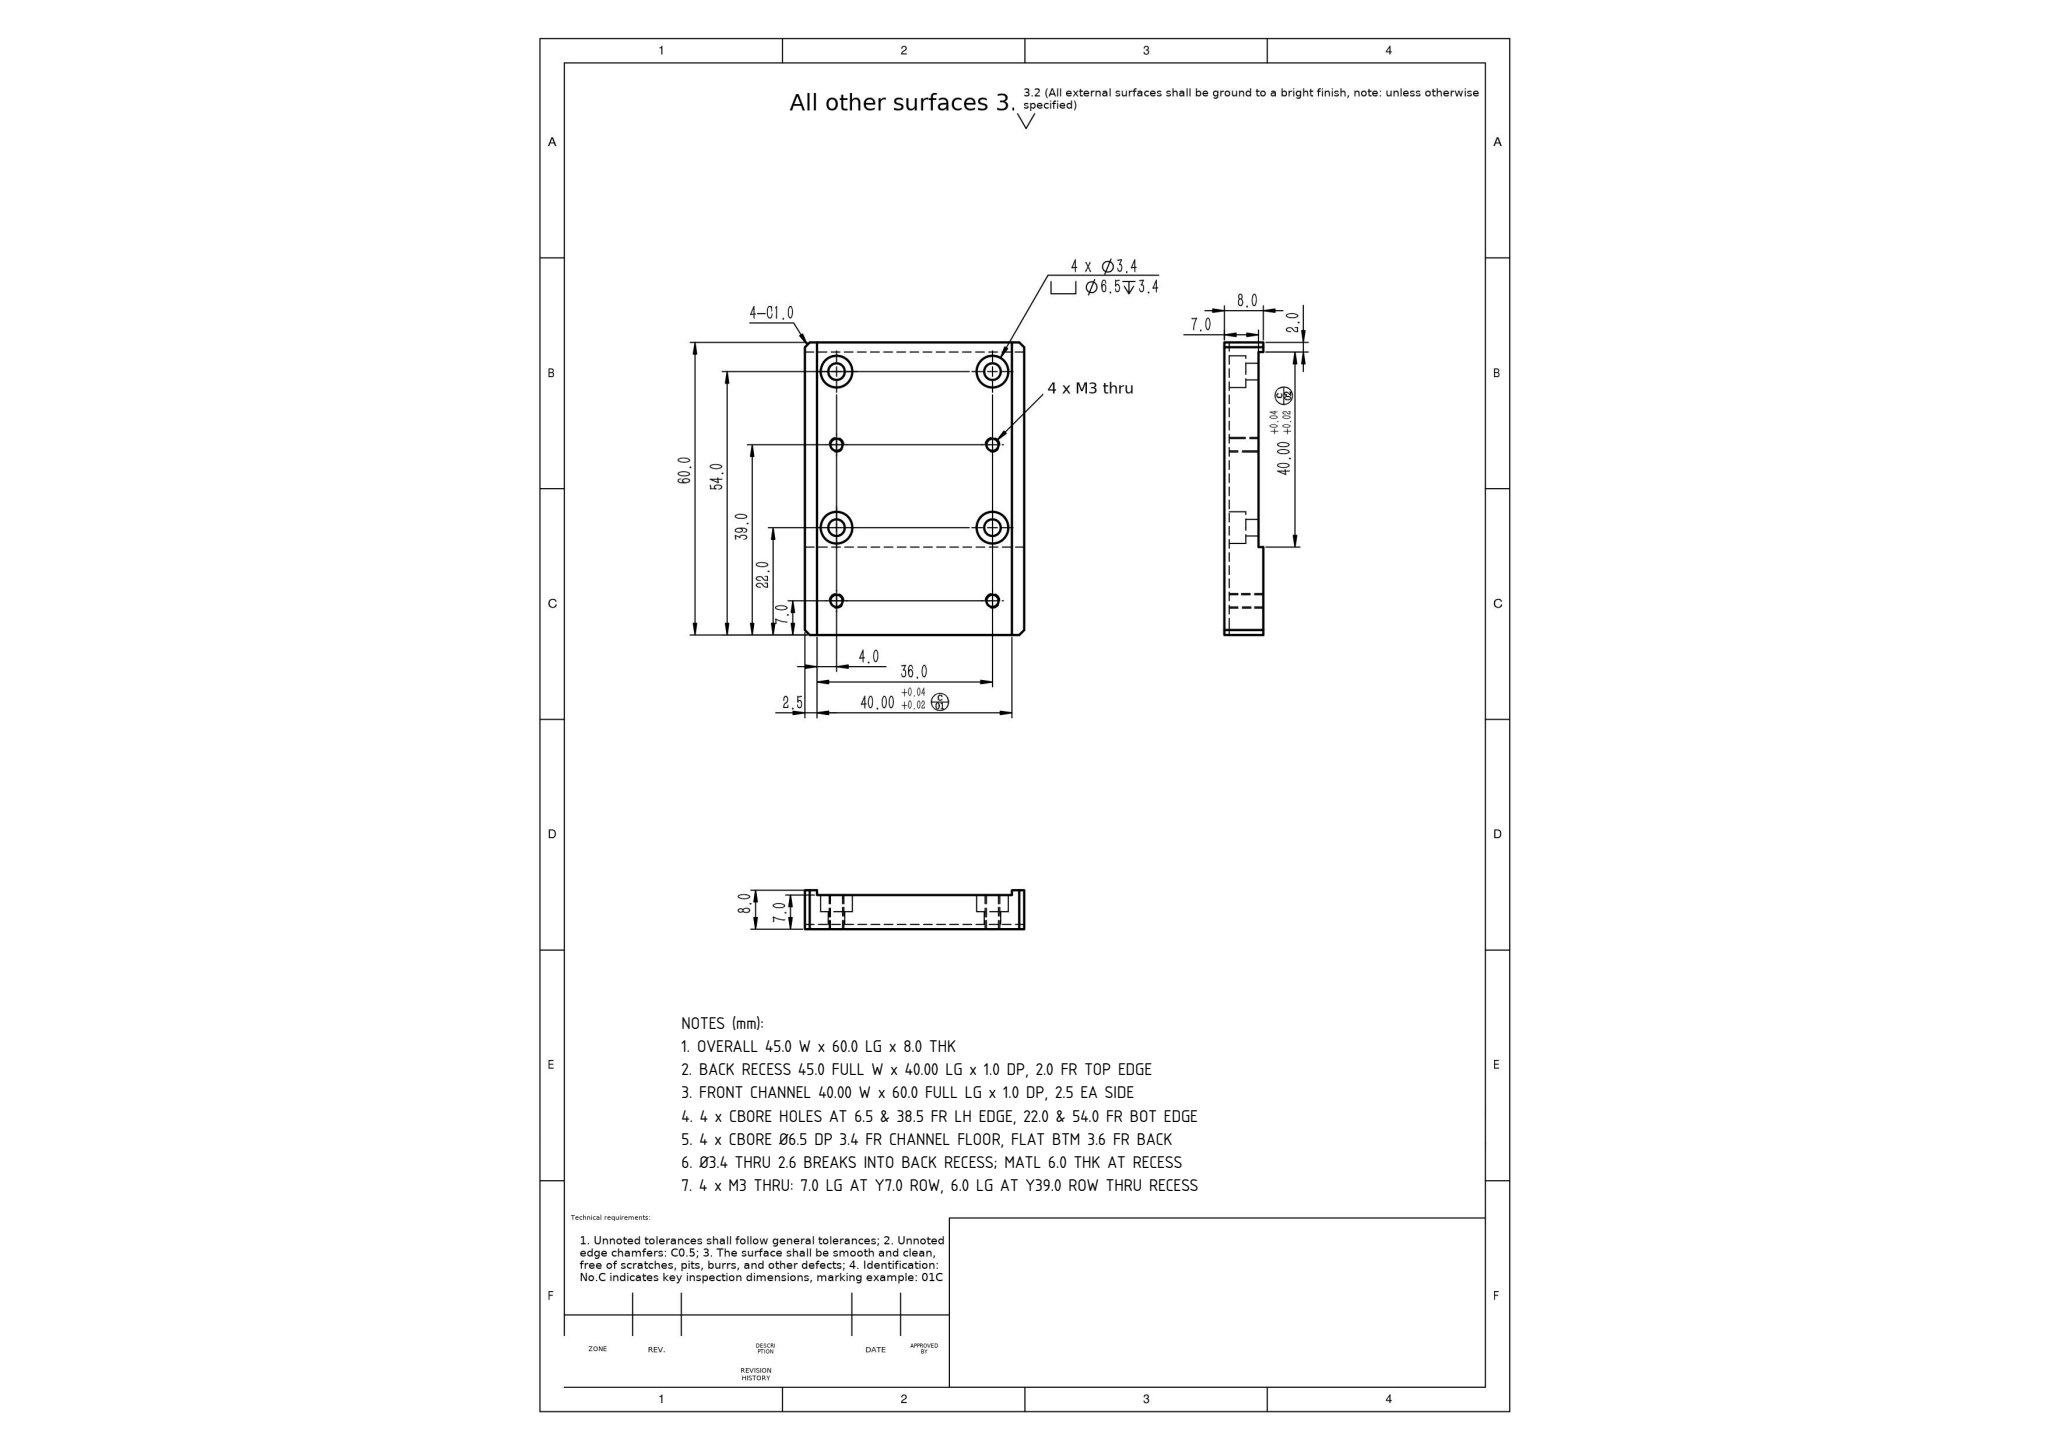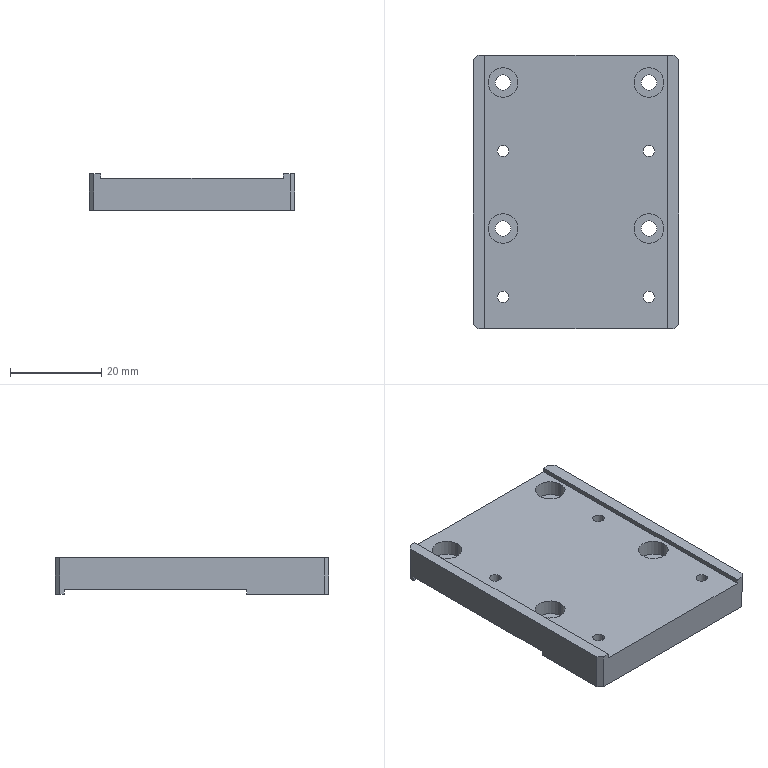Part | SolidWorks | mm | 1 solid | 46 faces | box 45 x 60 x 8 mm | volume 16711 mm3 | cylinder 24 | plane 22 | commonest cylinder face diameters 6.5 x8 3.4 x8 2.5 x8
Drawing notes:
OVERALL 45.0 W x 60.0 LG x 8.0 THK | from the solid: bbox_xyz 45.0 x 60.0 x 8.0
BACK RECESS 45.0 FULL W x 40.00 LG x 1.0 DP, 2.0 FR TOP EDGE | from the solid: y planes 18.0 & 58.0 (=40.00); 60-58=2.0; z plane 1.0 vs faces at z=0; full x 0-45
FRONT CHANNEL 40.00 W x 60.0 FULL LG x 1.0 DP, 2.5 EA SIDE | from the solid: x planes 2.5 & 42.5 (=40.00, 2.5 ea side of 45); z plane 7.0 vs faces at z=8.0
4 x CBORE HOLES AT 6.5 & 38.5 FR LH EDGE, 22.0 & 54.0 FR BOT EDGE | from the solid: Ø3.4/Ø6.5 axes at (6.5,22),(6.5,54),(38.5,22),(38.5,54)
4 x CBORE Ø6.5 DP 3.4 FR CHANNEL FLOOR, FLAT BTM 3.6 FR BACK | from the solid: Ø6.5 z-cyl len 3.4 from z=7.0; z-plane 3.6 count 4
Ø3.4 THRU 2.6 BREAKS INTO BACK RECESS; MATL 6.0 THK AT RECESS | from the solid: Ø3.4 len 2.6 from z=3.6 to z=1.0; recess floor z=1.0, channel floor z=7.0
4 x M3 THRU: 7.0 LG AT Y7.0 ROW, 6.0 LG AT Y39.0 ROW THRU RECESS | from the solid: Ø2.5 cyls len 7.0 at y=7.0, len 6.0 at y=39.0, x=6.5 & 38.5
build123d program:
from build123d import *

# Parameters (mm, degrees)
SKETCH1_W                                       = 45
SKETCH1_H                                       = 60
BOSS_EXTRUDE1_DEPTH                             = 8
SKETCH2_W                                       = 45
SKETCH2_H                                       = 40
CUT_EXTRUDE1_DEPTH                              = 1
SKETCH4_W                                       = 40
SKETCH4_H                                       = 2
CUT_EXTRUDE2_DEPTH                              = 65.577
M3_TAPPED_HOLE1_D                               = 2.5
M3_HEX_SOCKET_HEAD_CAP_SCREW_CBORE1_D           = 3.4
M3_HEX_SOCKET_HEAD_CAP_SCREW_CBORE1_CBORE_D     = 6.5
M3_HEX_SOCKET_HEAD_CAP_SCREW_CBORE1_CBORE_DEPTH = 3.4
CHAMFER1_SIZE                                   = 1


with BuildPart() as part:
    # Sketch1 → Boss-Extrude1 (new body)
    with BuildSketch(Plane.XY):
        Rectangle(SKETCH1_W, SKETCH1_H)
    extrude(amount=BOSS_EXTRUDE1_DEPTH)

    # Sketch2 → Cut-Extrude1 (cut)
    with BuildSketch(Plane(origin=(0, 0, 0), x_dir=(-1, 0, 0), z_dir=(0, 0, -1))):
        with Locations((0, 8)):
            Rectangle(SKETCH2_W, SKETCH2_H)
    extrude(amount=-CUT_EXTRUDE1_DEPTH, mode=Mode.SUBTRACT)

    # Sketch4 → Cut-Extrude2 (cut, through all)
    with BuildSketch(Plane.XZ.offset(30)):
        with Locations((0, 8)):
            Rectangle(SKETCH4_W, SKETCH4_H)
    extrude(amount=-CUT_EXTRUDE2_DEPTH, mode=Mode.SUBTRACT)

    # M3 Tapped Hole1 (through all)
    with Locations(Plane.XY.offset(7)):
        with Locations((-16, 9), (16, 9), (16, -23), (-16, -23)):
            Hole(M3_TAPPED_HOLE1_D / 2)

    # M3 Hex Socket Head Cap Screw CBORE1 (through all)
    with Locations(Plane.XY.offset(7)):
        with Locations((-16, -8), (-16, 24), (16, 24), (16, -8)):
            CounterBoreHole(M3_HEX_SOCKET_HEAD_CAP_SCREW_CBORE1_D / 2, M3_HEX_SOCKET_HEAD_CAP_SCREW_CBORE1_CBORE_D / 2, M3_HEX_SOCKET_HEAD_CAP_SCREW_CBORE1_CBORE_DEPTH)

    # Chamfer1
    chamfer1_edges = [part.edges().sort_by_distance(p)[0] for p in [
        (22.5, -30, 4),
        (-22.5, -30, 4),
        (-22.5, 30, 4),
        (22.5, 30, 4),
    ]]
    chamfer(chamfer1_edges, length=CHAMFER1_SIZE)


solid = part.part